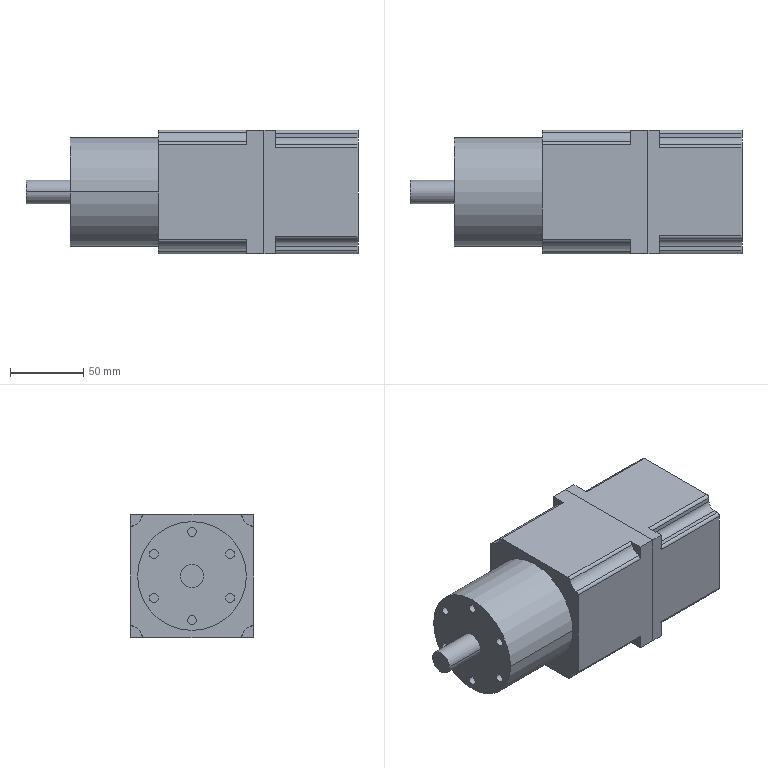Component | SolidWorks | TorqueMotor-1 | 2 solids | 106 faces | box 226 x 84 x 84 mm | volume 1185920 mm3 | cylinder 60 | plane 46 | commonest cylinder face diameters 4 x32 6 x12 16 x6 10 x4 74 x2 5.403 x2 5.5 x2
build123d program:
from build123d import *

# Parameters (mm, degrees)
SKETCH2_W            = 84
SKETCH2_H            = 84
BOSS_EXTRUDE1_DEPTH  = 72
SKETCH3_R            = 8
CUT_EXTRUDE1_2_DEPTH = 60
FILLET1_R            = 2
SKETCH4_R            = 2.702
BOSS_EXTRUDE2_DEPTH  = 20
CIRPATTERN2_COUNT    = 4
FILLET2_R            = 2
SKETCH5_R            = 2
CUT_EXTRUDE3_DEPTH   = 20
CIRPATTERN3_COUNT    = 4
SKETCH6_W            = 84
SKETCH6_H            = 84
BOSS_EXTRUDE3_DEPTH  = 64
CUT_EXTRUDE6_DEPTH   = 56
MIRROR5_COPY_1_DEPTH = 56
FILLET3_R            = 2
SKETCH11_R           = 37
BOSS_EXTRUDE5_DEPTH  = 60
SKETCH13_R           = 2
CUT_EXTRUDE7_DEPTH   = 30
CIRPATTERN8_COUNT    = 4
SKETCH14_R           = 8
BOSS_EXTRUDE6_DEPTH  = 30
SKETCH16_R           = 3
CUT_EXTRUDE8_DEPTH   = 10
CIRPATTERN9_COUNT    = 6
SKETCH1_R            = 2.75
CUT_EXTRUDE1_DEPTH   = 10.35


with BuildPart() as part:
    # Sketch2 → Boss-Extrude1 (new body)
    with BuildSketch(Plane.XY):
        Rectangle(SKETCH2_W, SKETCH2_H)
    extrude(amount=BOSS_EXTRUDE1_DEPTH)

    # Sketch3 → Cut-Extrude1_2 (cut)
    with BuildSketch(Plane(origin=(0, 0, 0), x_dir=(-1, 0, 0), z_dir=(0, 0, -1))):
        with Locations((-42, 42)):
            Circle(SKETCH3_R)
    cut_extrude1_2 = extrude(amount=-CUT_EXTRUDE1_2_DEPTH, mode=Mode.SUBTRACT)

    # Fillet1
    fillet1_edges = [part.edges().sort_by_distance(p)[0] for p in [
        (42, 34, 30),
        (34, 42, 30),
    ]]
    fillet(fillet1_edges, radius=FILLET1_R)

    # Sketch4 → Boss-Extrude2 (add)
    with BuildSketch(Plane.XY.offset(72)):
        with Locations(Location((0, 0, 0), (0, 0, 180))):
            Circle(SKETCH4_R)
    extrude(amount=BOSS_EXTRUDE2_DEPTH)

    # CirPattern2: Cut-Extrude1_2 ×4 about axis
    cirpattern2_axis = Axis((0, 0, 0), (0, 0, 1))
    for i in range(1, CIRPATTERN2_COUNT):
        add(cut_extrude1_2.rotate(cirpattern2_axis, i * 360 / CIRPATTERN2_COUNT), mode=Mode.SUBTRACT)

    # Fillet2
    fillet2_edges = [part.edges().sort_by_distance(p)[0] for p in [
        (42, -34, 30),
        (34, -42, 30),
        (-42, -34, 30),
        (-34, -42, 30),
        (-34, 42, 30),
        (-42, 34, 30),
    ]]
    fillet(fillet2_edges, radius=FILLET2_R)

    # Sketch5 → Cut-Extrude3 (cut)
    with BuildSketch(Plane(origin=(0, 0, 60), x_dir=(-1, 0, 0), z_dir=(0, 0, -1))):
        with Locations((17.678, 17.678)):
            Circle(SKETCH5_R)
    cut_extrude3 = extrude(amount=-CUT_EXTRUDE3_DEPTH, mode=Mode.SUBTRACT)

    # CirPattern3: Cut-Extrude3 ×4 about axis
    cirpattern3_axis = Axis((0, 0, 0), (0, 0, 1))
    for i in range(1, CIRPATTERN3_COUNT):
        add(cut_extrude3.rotate(cirpattern3_axis, i * 360 / CIRPATTERN3_COUNT), mode=Mode.SUBTRACT)

    # Sketch11 → Boss-Extrude5 (add)
    with BuildSketch(Plane(origin=(0, 0, 0), x_dir=(-1, 0, 0), z_dir=(0, 0, -1))):
        Circle(SKETCH11_R)
    extrude(amount=BOSS_EXTRUDE5_DEPTH)

    # Sketch14 → Boss-Extrude6 (add)
    with BuildSketch(Plane(origin=(0, 0, -60), x_dir=(-1, 0, 0), z_dir=(0, 0, -1))):
        Circle(SKETCH14_R)
    extrude(amount=BOSS_EXTRUDE6_DEPTH)

    # Sketch16 → Cut-Extrude8 (cut)
    with BuildSketch(Plane(origin=(0, 0, -60), x_dir=(-1, 0, 0), z_dir=(0, 0, -1))):
        with Locations((0, 30)):
            Circle(SKETCH16_R)
    cut_extrude8 = extrude(amount=-CUT_EXTRUDE8_DEPTH, mode=Mode.SUBTRACT)

    # CirPattern9: Cut-Extrude8 ×6 about axis
    cirpattern9_axis = Axis((0, 0, 0), (0, 0, 1))
    for i in range(1, CIRPATTERN9_COUNT):
        add(cut_extrude8.rotate(cirpattern9_axis, i * 360 / CIRPATTERN9_COUNT), mode=Mode.SUBTRACT)


with BuildPart() as body_2:
    # Sketch6 → Boss-Extrude3 (new body)
    with BuildSketch(Plane.XY.offset(72)):
        Rectangle(SKETCH6_W, SKETCH6_H)
    extrude(amount=BOSS_EXTRUDE3_DEPTH)

    # Sketch10 → Cut-Extrude6 (cut)
    with BuildSketch(Plane.XY.offset(136)):
        with BuildLine():
            Line((-32, 37), (-32, 42))
            Line((-32, 42), (-42, 42))
            Line((-42, 42), (-42, 32))
            Line((-42, 32), (-37, 32))
            ThreePointArc((-37, 32), (-33.464, 33.464), (-32, 37))
        make_face()
    cut_extrude6 = extrude(amount=-CUT_EXTRUDE6_DEPTH, mode=Mode.SUBTRACT)

    # Mirror4: Cut-Extrude6 across plane
    add(cut_extrude6.mirror(Plane.ZX), mode=Mode.SUBTRACT)

    # Mirror5: Cut-Extrude6 across plane
    add(cut_extrude6.mirror(Plane(origin=(0, 0, 0), x_dir=(0, 0, 1), z_dir=(1, 0, 0))), mode=Mode.SUBTRACT)

    # Mirror5 copy 1 sketch → Mirror5 copy 1 (cut)
    with BuildSketch(Plane(origin=(0, 0, 136), x_dir=(-1, 0, 0), z_dir=(0, 0, 1))):
        with BuildLine():
            Line((-32, 37), (-32, 42))
            Line((-32, 42), (-42, 42))
            Line((-42, 42), (-42, 32))
            Line((-42, 32), (-37, 32))
            ThreePointArc((-37, 32), (-33.464, 33.464), (-32, 37))
        make_face()
    extrude(amount=-MIRROR5_COPY_1_DEPTH, mode=Mode.SUBTRACT)

    # Fillet3
    fillet3_edges = [body_2.edges().sort_by_distance(p)[0] for p in [
        (-42, 32, 108),
        (-32, 42, 108),
        (-32, -42, 108),
        (-42, -32, 108),
        (42, -32, 108),
        (32, -42, 108),
        (32, 42, 108),
        (42, 32, 108),
    ]]
    fillet(fillet3_edges, radius=FILLET3_R)

    # Sketch13 → Cut-Extrude7 (cut)
    with BuildSketch(Plane(origin=(0, 0, 72), x_dir=(-1, 0, 0), z_dir=(0, 0, -1))):
        with Locations((17.678, 17.678)):
            Circle(SKETCH13_R)
    cut_extrude7 = extrude(amount=-CUT_EXTRUDE7_DEPTH, mode=Mode.SUBTRACT)

    # CirPattern8: Cut-Extrude7 ×4 about axis
    cirpattern8_axis = Axis((0, 0, 0), (0, 0, 1))
    for i in range(1, CIRPATTERN8_COUNT):
        add(cut_extrude7.rotate(cirpattern8_axis, i * 360 / CIRPATTERN8_COUNT), mode=Mode.SUBTRACT)

    # Sketch1 → Cut-Extrude1 (cut, symmetric)
    with BuildSketch(Plane.XY.offset(82.15)):
        Circle(SKETCH1_R)
    extrude(amount=CUT_EXTRUDE1_DEPTH, both=True, mode=Mode.SUBTRACT)


solid = Compound([part.part, body_2.part])

# Placed as in the assembly
solid = solid.moved(Location((-164.371, -367.407, 334), (90, 90, 0)))